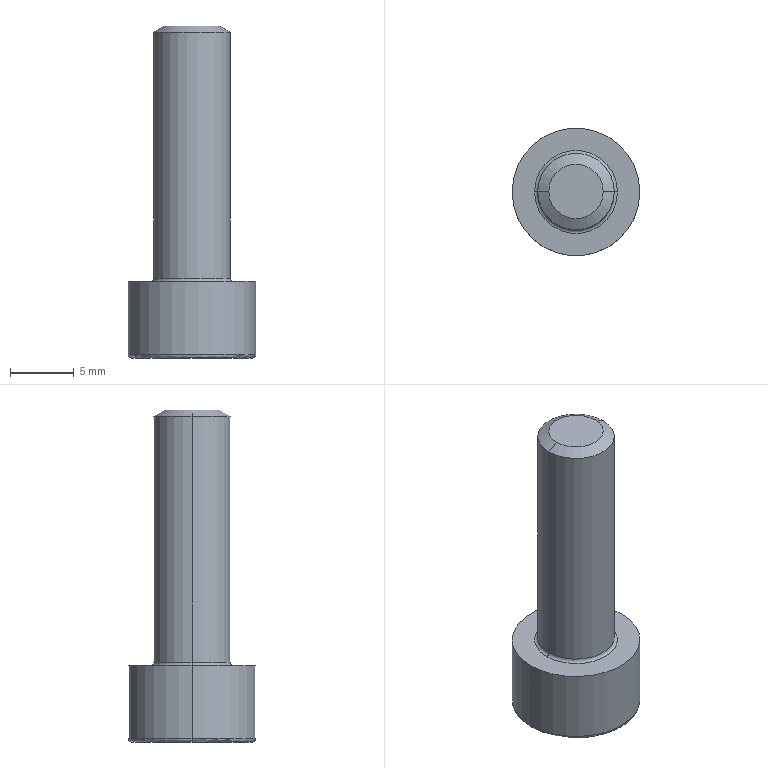Component | NX | SHCS_M6X20_4 | 1 solid | 20 faces | volume 969 mm3 | plane 10 | torus 4 | cylinder 4 | cone 2 | commonest cylinder face diameters 10 x2 6 x2